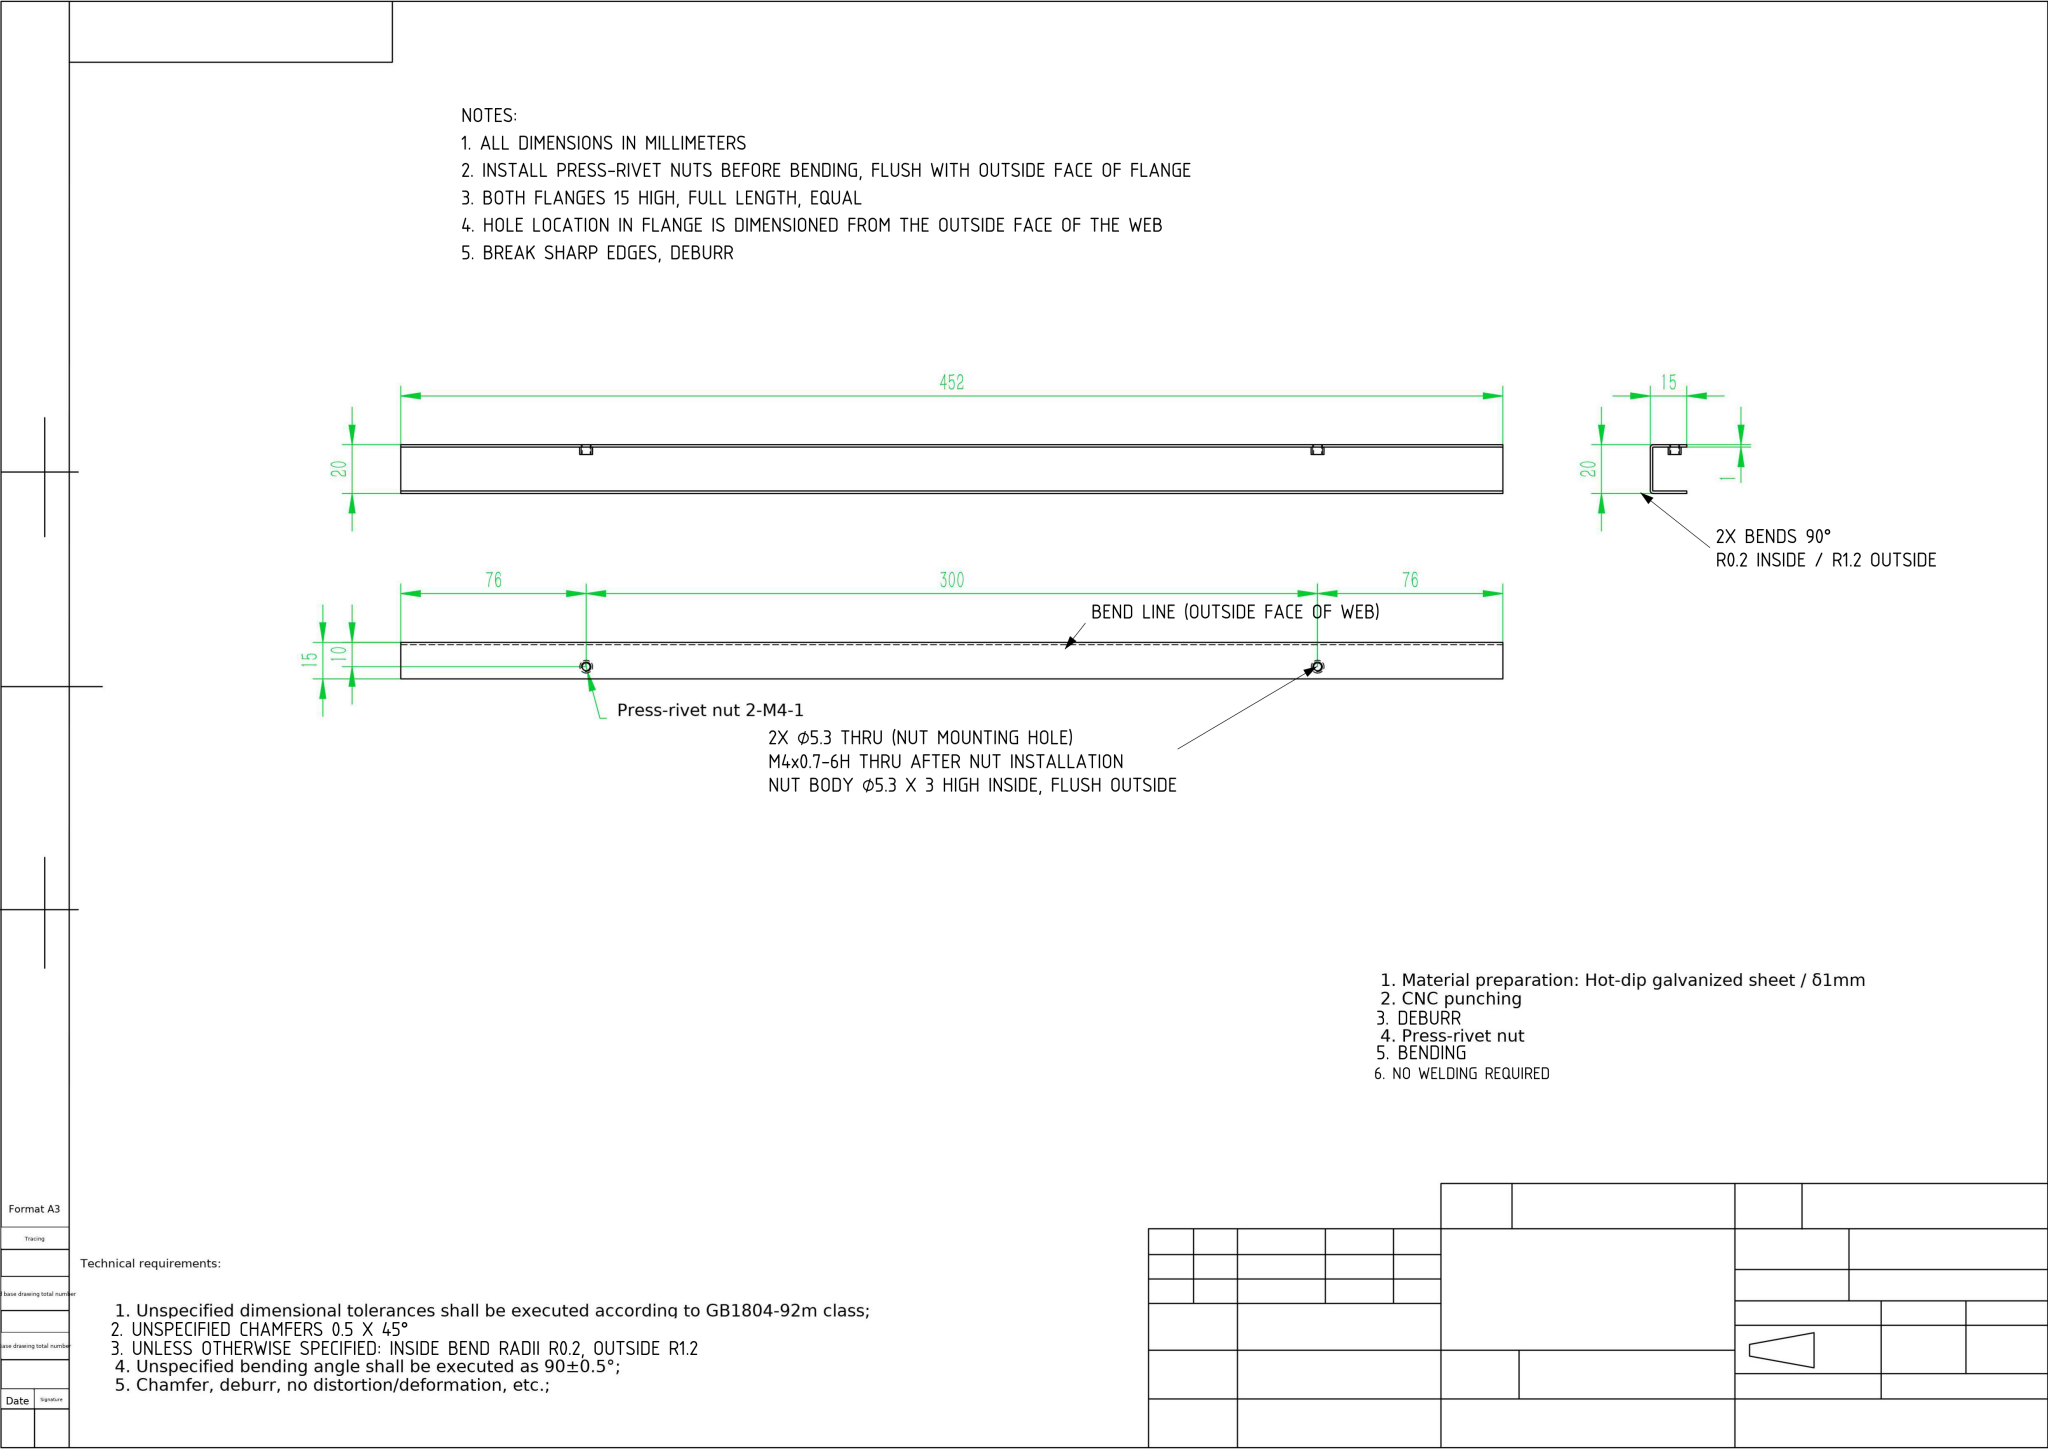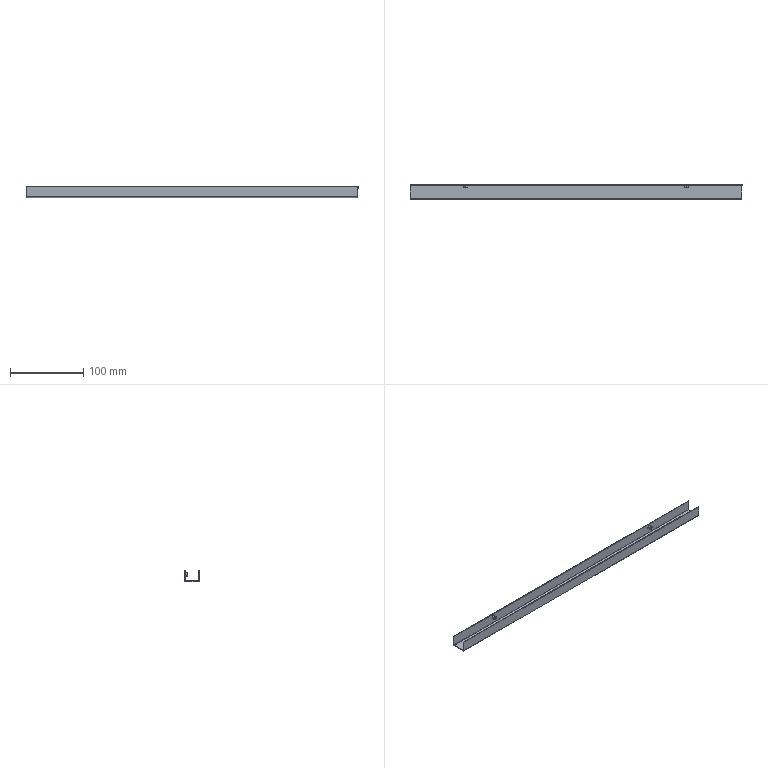Part | NX | mm | 1 solid | 32 faces | box 452 x 20 x 15 mm | volume 21488 mm3 | plane 20 | cylinder 12 | commonest cylinder face diameters 3.3 x4 5.3 x4 2.4 x2 0.4 x2
STEP:
#1=COLOUR_RGB('',0.7529,0.7529,0.7529);
#2=FILL_AREA_STYLE_COLOUR('',#1);
#3=FILL_AREA_STYLE('',(#2));
#4=SURFACE_STYLE_FILL_AREA(#3);
#5=SURFACE_SIDE_STYLE('',(#4));
#6=SURFACE_STYLE_USAGE(.BOTH.,#5);
#7=PRESENTATION_STYLE_ASSIGNMENT((#6));
#8=CARTESIAN_POINT('',(150.,6.,8.35));
#9=VERTEX_POINT('',#8);
#10=CARTESIAN_POINT('',(150.,10.,8.35));
#11=VERTEX_POINT('',#10);
#12=CARTESIAN_POINT('',(150.,10.,8.35));
#13=DIRECTION('',(-0.,1.,-0.));
#14=VECTOR('',#13,1000.);
#15=LINE('',#12,#14);
#16=EDGE_CURVE('',#9,#11,#15,.T.);
#17=ORIENTED_EDGE('',*,*,#16,.F.);
#18=CARTESIAN_POINT('',(150.,6.,11.65));
#19=VERTEX_POINT('',#18);
#20=CARTESIAN_POINT('',(150.,6.,10.));
#21=DIRECTION('',(-0.,1.,-0.));
#22=DIRECTION('',(0.,0.,1.));
#23=AXIS2_PLACEMENT_3D('',#20,#21,#22);
#24=CIRCLE('',#23,1.65);
#25=EDGE_CURVE('',#19,#9,#24,.T.);
#26=ORIENTED_EDGE('',*,*,#25,.F.);
#27=CARTESIAN_POINT('',(150.,10.,11.65));
#28=VERTEX_POINT('',#27);
#29=CARTESIAN_POINT('',(150.,10.,11.65));
#30=DIRECTION('',(-0.,1.,-0.));
#31=VECTOR('',#30,1000.);
#32=LINE('',#29,#31);
#33=EDGE_CURVE('',#19,#28,#32,.T.);
#34=ORIENTED_EDGE('',*,*,#33,.T.);
#35=CARTESIAN_POINT('',(150.,10.,10.));
#36=DIRECTION('',(-0.,1.,-0.));
#37=DIRECTION('',(0.,0.,1.));
#38=AXIS2_PLACEMENT_3D('',#35,#36,#37);
#39=CIRCLE('',#38,1.65);
#40=EDGE_CURVE('',#28,#11,#39,.T.);
#41=ORIENTED_EDGE('',*,*,#40,.T.);
#42=EDGE_LOOP('',(#17,#26,#34,#41));
#43=FACE_OUTER_BOUND('',#42,.T.);
#44=CARTESIAN_POINT('',(150.,10.,10.));
#45=DIRECTION('',(-0.,1.,-0.));
#46=DIRECTION('',(0.,0.,1.));
#47=AXIS2_PLACEMENT_3D('',#44,#45,#46);
#48=CYLINDRICAL_SURFACE('',#47,1.65);
#49=ADVANCED_FACE('',(#43),#48,.F.);
#50=STYLED_ITEM('',(#7),#49);
#51=PRESENTATION_LAYER_ASSIGNMENT('','',(#50));
#52=COLOUR_RGB('',0.7529,0.7529,0.7529);
#53=FILL_AREA_STYLE_COLOUR('',#52);
#54=FILL_AREA_STYLE('',(#53));
#55=SURFACE_STYLE_FILL_AREA(#54);
#56=SURFACE_SIDE_STYLE('',(#55));
#57=SURFACE_STYLE_USAGE(.BOTH.,#56);
#58=PRESENTATION_STYLE_ASSIGNMENT((#57));
#59=CARTESIAN_POINT('',(-150.,6.,8.35));
#60=VERTEX_POINT('',#59);
#61=CARTESIAN_POINT('',(-150.,10.,8.35));
#62=VERTEX_POINT('',#61);
#63=CARTESIAN_POINT('',(-150.,10.,8.35));
#64=DIRECTION('',(-0.,1.,-0.));
#65=VECTOR('',#64,1000.);
#66=LINE('',#63,#65);
#67=EDGE_CURVE('',#60,#62,#66,.T.);
#68=ORIENTED_EDGE('',*,*,#67,.F.);
#69=CARTESIAN_POINT('',(-150.,6.,11.65));
#70=VERTEX_POINT('',#69);
#71=CARTESIAN_POINT('',(-150.,6.,10.));
#72=DIRECTION('',(-0.,1.,-0.));
#73=DIRECTION('',(0.,0.,1.));
#74=AXIS2_PLACEMENT_3D('',#71,#72,#73);
#75=CIRCLE('',#74,1.65);
#76=EDGE_CURVE('',#70,#60,#75,.T.);
#77=ORIENTED_EDGE('',*,*,#76,.F.);
#78=CARTESIAN_POINT('',(-150.,10.,11.65));
#79=VERTEX_POINT('',#78);
#80=CARTESIAN_POINT('',(-150.,10.,11.65));
#81=DIRECTION('',(-0.,1.,-0.));
#82=VECTOR('',#81,1000.);
#83=LINE('',#80,#82);
#84=EDGE_CURVE('',#70,#79,#83,.T.);
#85=ORIENTED_EDGE('',*,*,#84,.T.);
#86=CARTESIAN_POINT('',(-150.,10.,10.));
#87=DIRECTION('',(-0.,1.,-0.));
#88=DIRECTION('',(0.,0.,1.));
#89=AXIS2_PLACEMENT_3D('',#86,#87,#88);
#90=CIRCLE('',#89,1.65);
#91=EDGE_CURVE('',#79,#62,#90,.T.);
#92=ORIENTED_EDGE('',*,*,#91,.T.);
#93=EDGE_LOOP('',(#68,#77,#85,#92));
#94=FACE_OUTER_BOUND('',#93,.T.);
#95=CARTESIAN_POINT('',(-150.,10.,10.));
#96=DIRECTION('',(-0.,1.,-0.));
#97=DIRECTION('',(0.,0.,1.));
#98=AXIS2_PLACEMENT_3D('',#95,#96,#97);
#99=CYLINDRICAL_SURFACE('',#98,1.65);
#100=ADVANCED_FACE('',(#94),#99,.F.);
#101=STYLED_ITEM('',(#58),#100);
#102=(LENGTH_UNIT()NAMED_UNIT(*)SI_UNIT(.MILLI.,.METRE.));
#103=UNCERTAINTY_MEASURE_WITH_UNIT(LENGTH_MEASURE(0.00001),#102,'','');
#104=(NAMED_UNIT(*)PLANE_ANGLE_UNIT()SI_UNIT($,.RADIAN.));
#105=(NAMED_UNIT(*)SI_UNIT($,.STERADIAN.)SOLID_ANGLE_UNIT());
#106=(GEOMETRIC_REPRESENTATION_CONTEXT(3)GLOBAL_UNCERTAINTY_ASSIGNED_CONTEXT((#103))GLOBAL_UNIT_ASSIGNED_CONTEXT((#102,#104,#105))REPRESENTATION_CONTEXT('',''));
#107=MECHANICAL_DESIGN_GEOMETRIC_PRESENTATION_REPRESENTATION('',(#101),#106);
#108=COLOUR_RGB('',0.7529,0.7529,0.7529);
#109=FILL_AREA_STYLE_COLOUR('',#108);
#110=FILL_AREA_STYLE('',(#109));
#111=SURFACE_STYLE_FILL_AREA(#110);
#112=SURFACE_SIDE_STYLE('',(#111));
#113=SURFACE_STYLE_USAGE(.BOTH.,#112);
#114=PRESENTATION_STYLE_ASSIGNMENT((#113));
#115=CARTESIAN_POINT('',(-150.,6.,10.));
#116=DIRECTION('',(-0.,1.,-0.));
#117=DIRECTION('',(0.,0.,1.));
#118=AXIS2_PLACEMENT_3D('',#115,#116,#117);
#119=CIRCLE('',#118,1.65);
#120=EDGE_CURVE('',#60,#70,#119,.T.);
#121=ORIENTED_EDGE('',*,*,#120,.F.);
#122=ORIENTED_EDGE('',*,*,#67,.T.);
#123=CARTESIAN_POINT('',(-150.,10.,10.));
#124=DIRECTION('',(-0.,1.,-0.));
#125=DIRECTION('',(0.,0.,1.));
#126=AXIS2_PLACEMENT_3D('',#123,#124,#125);
#127=CIRCLE('',#126,1.65);
#128=EDGE_CURVE('',#62,#79,#127,.T.);
#129=ORIENTED_EDGE('',*,*,#128,.T.);
#130=ORIENTED_EDGE('',*,*,#84,.F.);
#131=EDGE_LOOP('',(#121,#122,#129,#130));
#132=FACE_OUTER_BOUND('',#131,.T.);
#133=CARTESIAN_POINT('',(-150.,10.,10.));
#134=DIRECTION('',(-0.,1.,-0.));
#135=DIRECTION('',(0.,0.,1.));
#136=AXIS2_PLACEMENT_3D('',#133,#134,#135);
#137=CYLINDRICAL_SURFACE('',#136,1.65);
#138=ADVANCED_FACE('',(#132),#137,.F.);
#139=STYLED_ITEM('',(#114),#138);
#140=PRESENTATION_LAYER_ASSIGNMENT('','',(#139));
#141=COLOUR_RGB('',0.7529,0.7529,0.7529);
#142=FILL_AREA_STYLE_COLOUR('',#141);
#143=FILL_AREA_STYLE('',(#142));
#144=SURFACE_STYLE_FILL_AREA(#143);
#145=SURFACE_SIDE_STYLE('',(#144));
#146=SURFACE_STYLE_USAGE(.BOTH.,#145);
#147=PRESENTATION_STYLE_ASSIGNMENT((#146));
#148=CARTESIAN_POINT('',(150.,6.,10.));
#149=DIRECTION('',(-0.,1.,-0.));
#150=DIRECTION('',(0.,0.,1.));
#151=AXIS2_PLACEMENT_3D('',#148,#149,#150);
#152=CIRCLE('',#151,1.65);
#153=EDGE_CURVE('',#9,#19,#152,.T.);
#154=ORIENTED_EDGE('',*,*,#153,.F.);
#155=ORIENTED_EDGE('',*,*,#16,.T.);
#156=CARTESIAN_POINT('',(150.,10.,10.));
#157=DIRECTION('',(-0.,1.,-0.));
#158=DIRECTION('',(0.,0.,1.));
#159=AXIS2_PLACEMENT_3D('',#156,#157,#158);
#160=CIRCLE('',#159,1.65);
#161=EDGE_CURVE('',#11,#28,#160,.T.);
#162=ORIENTED_EDGE('',*,*,#161,.T.);
#163=ORIENTED_EDGE('',*,*,#33,.F.);
#164=EDGE_LOOP('',(#154,#155,#162,#163));
#165=FACE_OUTER_BOUND('',#164,.T.);
#166=CARTESIAN_POINT('',(150.,10.,10.));
#167=DIRECTION('',(-0.,1.,-0.));
#168=DIRECTION('',(0.,0.,1.));
#169=AXIS2_PLACEMENT_3D('',#166,#167,#168);
#170=CYLINDRICAL_SURFACE('',#169,1.65);
#171=ADVANCED_FACE('',(#165),#170,.F.);
#172=CARTESIAN_POINT('',(150.,6.,7.35));
#173=VERTEX_POINT('',#172);
#174=CARTESIAN_POINT('',(150.,6.,12.65));
#175=VERTEX_POINT('',#174);
#176=CARTESIAN_POINT('',(150.,6.,10.));
#177=DIRECTION('',(0.,-1.,0.));
#178=DIRECTION('',(0.,0.,1.));
#179=AXIS2_PLACEMENT_3D('',#176,#177,#178);
#180=CIRCLE('',#179,2.65);
#181=EDGE_CURVE('',#173,#175,#180,.T.);
#182=ORIENTED_EDGE('',*,*,#181,.F.);
#183=CARTESIAN_POINT('',(150.,9.,7.35));
#184=VERTEX_POINT('',#183);
#185=CARTESIAN_POINT('',(150.,6.,7.35));
#186=DIRECTION('',(-0.,1.,-0.));
#187=VECTOR('',#186,1000.);
#188=LINE('',#185,#187);
#189=EDGE_CURVE('',#173,#184,#188,.T.);
#190=ORIENTED_EDGE('',*,*,#189,.T.);
#191=CARTESIAN_POINT('',(150.,9.,12.65));
#192=VERTEX_POINT('',#191);
#193=CARTESIAN_POINT('',(150.,9.,10.));
#194=DIRECTION('',(0.,-1.,0.));
#195=DIRECTION('',(0.,0.,1.));
#196=AXIS2_PLACEMENT_3D('',#193,#194,#195);
#197=CIRCLE('',#196,2.65);
#198=EDGE_CURVE('',#184,#192,#197,.T.);
#199=ORIENTED_EDGE('',*,*,#198,.T.);
#200=CARTESIAN_POINT('',(150.,6.,12.65));
#201=DIRECTION('',(-0.,1.,-0.));
#202=VECTOR('',#201,1000.);
#203=LINE('',#200,#202);
#204=EDGE_CURVE('',#175,#192,#203,.T.);
#205=ORIENTED_EDGE('',*,*,#204,.F.);
#206=EDGE_LOOP('',(#182,#190,#199,#205));
#207=FACE_OUTER_BOUND('',#206,.T.);
#208=CARTESIAN_POINT('',(150.,6.,10.));
#209=DIRECTION('',(-0.,1.,-0.));
#210=DIRECTION('',(0.,0.,1.));
#211=AXIS2_PLACEMENT_3D('',#208,#209,#210);
#212=CYLINDRICAL_SURFACE('',#211,2.65);
#213=ADVANCED_FACE('',(#207),#212,.T.);
#214=CARTESIAN_POINT('',(-150.,6.,12.65));
#215=VERTEX_POINT('',#214);
#216=CARTESIAN_POINT('',(-150.,6.,7.35));
#217=VERTEX_POINT('',#216);
#218=CARTESIAN_POINT('',(-150.,6.,10.));
#219=DIRECTION('',(-0.,1.,-0.));
#220=DIRECTION('',(0.,0.,1.));
#221=AXIS2_PLACEMENT_3D('',#218,#219,#220);
#222=CIRCLE('',#221,2.65);
#223=EDGE_CURVE('',#215,#217,#222,.T.);
#224=ORIENTED_EDGE('',*,*,#223,.T.);
#225=CARTESIAN_POINT('',(-150.,9.,7.35));
#226=VERTEX_POINT('',#225);
#227=CARTESIAN_POINT('',(-150.,6.,7.35));
#228=DIRECTION('',(-0.,1.,-0.));
#229=VECTOR('',#228,1000.);
#230=LINE('',#227,#229);
#231=EDGE_CURVE('',#217,#226,#230,.T.);
#232=ORIENTED_EDGE('',*,*,#231,.T.);
#233=CARTESIAN_POINT('',(-150.,9.,12.65));
#234=VERTEX_POINT('',#233);
#235=CARTESIAN_POINT('',(-150.,9.,10.));
#236=DIRECTION('',(-0.,1.,-0.));
#237=DIRECTION('',(0.,0.,1.));
#238=AXIS2_PLACEMENT_3D('',#235,#236,#237);
#239=CIRCLE('',#238,2.65);
#240=EDGE_CURVE('',#234,#226,#239,.T.);
#241=ORIENTED_EDGE('',*,*,#240,.F.);
#242=CARTESIAN_POINT('',(-150.,6.,12.65));
#243=DIRECTION('',(-0.,1.,-0.));
#244=VECTOR('',#243,1000.);
#245=LINE('',#242,#244);
#246=EDGE_CURVE('',#215,#234,#245,.T.);
#247=ORIENTED_EDGE('',*,*,#246,.F.);
#248=EDGE_LOOP('',(#224,#232,#241,#247));
#249=FACE_OUTER_BOUND('',#248,.T.);
#250=CARTESIAN_POINT('',(-150.,6.,10.));
#251=DIRECTION('',(-0.,1.,-0.));
#252=DIRECTION('',(0.,0.,1.));
#253=AXIS2_PLACEMENT_3D('',#250,#251,#252);
#254=CYLINDRICAL_SURFACE('',#253,2.65);
#255=ADVANCED_FACE('',(#249),#254,.T.);
#256=CARTESIAN_POINT('',(226.,9.,1.2));
#257=VERTEX_POINT('',#256);
#258=CARTESIAN_POINT('',(-226.,9.,1.2));
#259=VERTEX_POINT('',#258);
#260=CARTESIAN_POINT('',(226.,9.,1.2));
#261=DIRECTION('',(-1.,0.,0.));
#262=VECTOR('',#261,1000.);
#263=LINE('',#260,#262);
#264=EDGE_CURVE('',#257,#259,#263,.T.);
#265=ORIENTED_EDGE('',*,*,#264,.F.);
#266=CARTESIAN_POINT('',(226.,9.,15.));
#267=VERTEX_POINT('',#266);
#268=CARTESIAN_POINT('',(226.,9.,-0.));
#269=DIRECTION('',(-0.,0.,1.));
#270=VECTOR('',#269,1000.);
#271=LINE('',#268,#270);
#272=EDGE_CURVE('',#257,#267,#271,.T.);
#273=ORIENTED_EDGE('',*,*,#272,.T.);
#274=CARTESIAN_POINT('',(-226.,9.,15.));
#275=VERTEX_POINT('',#274);
#276=CARTESIAN_POINT('',(0.,9.,15.));
#277=DIRECTION('',(-1.,0.,0.));
#278=VECTOR('',#277,1000.);
#279=LINE('',#276,#278);
#280=EDGE_CURVE('',#267,#275,#279,.T.);
#281=ORIENTED_EDGE('',*,*,#280,.T.);
#282=CARTESIAN_POINT('',(-226.,9.,0.));
#283=DIRECTION('',(0.,-0.,-1.));
#284=VECTOR('',#283,1000.);
#285=LINE('',#282,#284);
#286=EDGE_CURVE('',#275,#259,#285,.T.);
#287=ORIENTED_EDGE('',*,*,#286,.T.);
#288=EDGE_LOOP('',(#265,#273,#281,#287));
#289=FACE_OUTER_BOUND('',#288,.T.);
#290=ORIENTED_EDGE('',*,*,#240,.T.);
#291=CARTESIAN_POINT('',(-150.,9.,10.));
#292=DIRECTION('',(-0.,1.,-0.));
#293=DIRECTION('',(0.,0.,1.));
#294=AXIS2_PLACEMENT_3D('',#291,#292,#293);
#295=CIRCLE('',#294,2.65);
#296=EDGE_CURVE('',#226,#234,#295,.T.);
#297=ORIENTED_EDGE('',*,*,#296,.T.);
#298=EDGE_LOOP('',(#290,#297));
#299=FACE_BOUND('',#298,.T.);
#300=CARTESIAN_POINT('',(150.,9.,10.));
#301=DIRECTION('',(0.,-1.,0.));
#302=DIRECTION('',(0.,0.,1.));
#303=AXIS2_PLACEMENT_3D('',#300,#301,#302);
#304=CIRCLE('',#303,2.65);
#305=EDGE_CURVE('',#192,#184,#304,.T.);
#306=ORIENTED_EDGE('',*,*,#305,.F.);
#307=ORIENTED_EDGE('',*,*,#198,.F.);
#308=EDGE_LOOP('',(#306,#307));
#309=FACE_BOUND('',#308,.T.);
#310=CARTESIAN_POINT('',(-0.,9.,0.));
#311=DIRECTION('',(-0.,1.,-0.));
#312=DIRECTION('',(-0.,0.,1.));
#313=AXIS2_PLACEMENT_3D('',#310,#311,#312);
#314=PLANE('',#313);
#315=ADVANCED_FACE('',(#289,#299,#309),#314,.F.);
#316=CARTESIAN_POINT('',(-226.,-8.8,1.));
#317=VERTEX_POINT('',#316);
#318=CARTESIAN_POINT('',(-226.,-8.8,0.));
#319=VERTEX_POINT('',#318);
#320=CARTESIAN_POINT('',(-226.,-8.8,1.));
#321=DIRECTION('',(0.,0.,-1.));
#322=VECTOR('',#321,1000.);
#323=LINE('',#320,#322);
#324=EDGE_CURVE('',#317,#319,#323,.T.);
#325=ORIENTED_EDGE('',*,*,#324,.F.);
#326=CARTESIAN_POINT('',(-226.,8.8,1.));
#327=VERTEX_POINT('',#326);
#328=CARTESIAN_POINT('',(-226.,10.,1.));
#329=DIRECTION('',(0.,-1.,-0.));
#330=VECTOR('',#329,1000.);
#331=LINE('',#328,#330);
#332=EDGE_CURVE('',#327,#317,#331,.T.);
#333=ORIENTED_EDGE('',*,*,#332,.F.);
#334=CARTESIAN_POINT('',(-226.,8.8,0.));
#335=VERTEX_POINT('',#334);
#336=CARTESIAN_POINT('',(-226.,8.8,1.));
#337=DIRECTION('',(0.,-0.,-1.));
#338=VECTOR('',#337,1000.);
#339=LINE('',#336,#338);
#340=EDGE_CURVE('',#327,#335,#339,.T.);
#341=ORIENTED_EDGE('',*,*,#340,.T.);
#342=CARTESIAN_POINT('',(-226.,10.,0.));
#343=DIRECTION('',(0.,-1.,-0.));
#344=VECTOR('',#343,1000.);
#345=LINE('',#342,#344);
#346=EDGE_CURVE('',#335,#319,#345,.T.);
#347=ORIENTED_EDGE('',*,*,#346,.T.);
#348=EDGE_LOOP('',(#325,#333,#341,#347));
#349=FACE_OUTER_BOUND('',#348,.T.);
#350=CARTESIAN_POINT('',(-226.,10.,1.));
#351=DIRECTION('',(1.,-0.,0.));
#352=DIRECTION('',(0.,-0.,-1.));
#353=AXIS2_PLACEMENT_3D('',#350,#351,#352);
#354=PLANE('',#353);
#355=ADVANCED_FACE('',(#349),#354,.F.);
#356=CARTESIAN_POINT('',(226.,-8.8,1.));
#357=VERTEX_POINT('',#356);
#358=CARTESIAN_POINT('',(226.,-8.8,-0.));
#359=VERTEX_POINT('',#358);
#360=CARTESIAN_POINT('',(226.,-8.8,1.));
#361=DIRECTION('',(0.,0.,-1.));
#362=VECTOR('',#361,1000.);
#363=LINE('',#360,#362);
#364=EDGE_CURVE('',#357,#359,#363,.T.);
#365=ORIENTED_EDGE('',*,*,#364,.T.);
#366=CARTESIAN_POINT('',(226.,8.8,-0.));
#367=VERTEX_POINT('',#366);
#368=CARTESIAN_POINT('',(226.,10.,-0.));
#369=DIRECTION('',(-0.,1.,0.));
#370=VECTOR('',#369,1000.);
#371=LINE('',#368,#370);
#372=EDGE_CURVE('',#359,#367,#371,.T.);
#373=ORIENTED_EDGE('',*,*,#372,.T.);
#374=CARTESIAN_POINT('',(226.,8.8,1.));
#375=VERTEX_POINT('',#374);
#376=CARTESIAN_POINT('',(226.,8.8,1.));
#377=DIRECTION('',(0.,-0.,-1.));
#378=VECTOR('',#377,1000.);
#379=LINE('',#376,#378);
#380=EDGE_CURVE('',#375,#367,#379,.T.);
#381=ORIENTED_EDGE('',*,*,#380,.F.);
#382=CARTESIAN_POINT('',(226.,10.,1.));
#383=DIRECTION('',(-0.,1.,0.));
#384=VECTOR('',#383,1000.);
#385=LINE('',#382,#384);
#386=EDGE_CURVE('',#357,#375,#385,.T.);
#387=ORIENTED_EDGE('',*,*,#386,.F.);
#388=EDGE_LOOP('',(#365,#373,#381,#387));
#389=FACE_OUTER_BOUND('',#388,.T.);
#390=CARTESIAN_POINT('',(226.,10.,1.));
#391=DIRECTION('',(-1.,0.,-0.));
#392=DIRECTION('',(-0.,0.,1.));
#393=AXIS2_PLACEMENT_3D('',#390,#391,#392);
#394=PLANE('',#393);
#395=ADVANCED_FACE('',(#389),#394,.F.);
#396=CARTESIAN_POINT('',(226.,-8.8,1.));
#397=DIRECTION('',(-1.,0.,0.));
#398=VECTOR('',#397,1000.);
#399=LINE('',#396,#398);
#400=EDGE_CURVE('',#357,#317,#399,.T.);
#401=ORIENTED_EDGE('',*,*,#400,.F.);
#402=ORIENTED_EDGE('',*,*,#386,.T.);
#403=CARTESIAN_POINT('',(-226.,8.8,1.));
#404=DIRECTION('',(1.,-0.,-0.));
#405=VECTOR('',#404,1000.);
#406=LINE('',#403,#405);
#407=EDGE_CURVE('',#327,#375,#406,.T.);
#408=ORIENTED_EDGE('',*,*,#407,.F.);
#409=ORIENTED_EDGE('',*,*,#332,.T.);
#410=EDGE_LOOP('',(#401,#402,#408,#409));
#411=FACE_OUTER_BOUND('',#410,.T.);
#412=CARTESIAN_POINT('',(0.,0.,1.));
#413=DIRECTION('',(-0.,-0.,-1.));
#414=DIRECTION('',(-1.,0.,0.));
#415=AXIS2_PLACEMENT_3D('',#412,#413,#414);
#416=PLANE('',#415);
#417=ADVANCED_FACE('',(#411),#416,.F.);
#418=ORIENTED_EDGE('',*,*,#372,.F.);
#419=CARTESIAN_POINT('',(226.,-8.8,-0.));
#420=DIRECTION('',(-1.,0.,0.));
#421=VECTOR('',#420,1000.);
#422=LINE('',#419,#421);
#423=EDGE_CURVE('',#359,#319,#422,.T.);
#424=ORIENTED_EDGE('',*,*,#423,.T.);
#425=ORIENTED_EDGE('',*,*,#346,.F.);
#426=CARTESIAN_POINT('',(-226.,8.8,0.));
#427=DIRECTION('',(1.,-0.,-0.));
#428=VECTOR('',#427,1000.);
#429=LINE('',#426,#428);
#430=EDGE_CURVE('',#335,#367,#429,.T.);
#431=ORIENTED_EDGE('',*,*,#430,.T.);
#432=EDGE_LOOP('',(#418,#424,#425,#431));
#433=FACE_OUTER_BOUND('',#432,.T.);
#434=CARTESIAN_POINT('',(0.,0.,0.));
#435=DIRECTION('',(-0.,-0.,-1.));
#436=DIRECTION('',(-1.,0.,0.));
#437=AXIS2_PLACEMENT_3D('',#434,#435,#436);
#438=PLANE('',#437);
#439=ADVANCED_FACE('',(#433),#438,.T.);
#440=CARTESIAN_POINT('',(226.,10.,1.2));
#441=VERTEX_POINT('',#440);
#442=CARTESIAN_POINT('',(226.,10.,1.2));
#443=DIRECTION('',(-0.,1.,-0.));
#444=VECTOR('',#443,1000.);
#445=LINE('',#442,#444);
#446=EDGE_CURVE('',#257,#441,#445,.T.);
#447=ORIENTED_EDGE('',*,*,#446,.F.);
#448=CARTESIAN_POINT('',(226.,8.8,1.2));
#449=DIRECTION('',(1.,-0.,-0.));
#450=DIRECTION('',(0.,0.,1.));
#451=AXIS2_PLACEMENT_3D('',#448,#449,#450);
#452=CIRCLE('',#451,0.2);
#453=EDGE_CURVE('',#375,#257,#452,.T.);
#454=ORIENTED_EDGE('',*,*,#453,.F.);
#455=ORIENTED_EDGE('',*,*,#380,.T.);
#456=CARTESIAN_POINT('',(226.,8.8,1.2));
#457=DIRECTION('',(1.,-0.,-0.));
#458=DIRECTION('',(0.,0.,1.));
#459=AXIS2_PLACEMENT_3D('',#456,#457,#458);
#460=CIRCLE('',#459,1.2);
#461=EDGE_CURVE('',#367,#441,#460,.T.);
#462=ORIENTED_EDGE('',*,*,#461,.T.);
#463=EDGE_LOOP('',(#447,#454,#455,#462));
#464=FACE_OUTER_BOUND('',#463,.T.);
#465=CARTESIAN_POINT('',(226.,8.8,1.2));
#466=DIRECTION('',(1.,-0.,0.));
#467=DIRECTION('',(0.,-0.,-1.));
#468=AXIS2_PLACEMENT_3D('',#465,#466,#467);
#469=PLANE('',#468);
#470=ADVANCED_FACE('',(#464),#469,.T.);
#471=CARTESIAN_POINT('',(-226.,8.8,1.2));
#472=DIRECTION('',(-1.,0.,0.));
#473=DIRECTION('',(0.,0.,1.));
#474=AXIS2_PLACEMENT_3D('',#471,#472,#473);
#475=CIRCLE('',#474,0.2);
#476=EDGE_CURVE('',#259,#327,#475,.T.);
#477=ORIENTED_EDGE('',*,*,#476,.F.);
#478=CARTESIAN_POINT('',(-226.,10.,1.2));
#479=VERTEX_POINT('',#478);
#480=CARTESIAN_POINT('',(-226.,9.,1.2));
#481=DIRECTION('',(-0.,1.,-0.));
#482=VECTOR('',#481,1000.);
#483=LINE('',#480,#482);
#484=EDGE_CURVE('',#259,#479,#483,.T.);
#485=ORIENTED_EDGE('',*,*,#484,.T.);
#486=CARTESIAN_POINT('',(-226.,8.8,1.2));
#487=DIRECTION('',(-1.,0.,0.));
#488=DIRECTION('',(0.,0.,1.));
#489=AXIS2_PLACEMENT_3D('',#486,#487,#488);
#490=CIRCLE('',#489,1.2);
#491=EDGE_CURVE('',#479,#335,#490,.T.);
#492=ORIENTED_EDGE('',*,*,#491,.T.);
#493=ORIENTED_EDGE('',*,*,#340,.F.);
#494=EDGE_LOOP('',(#477,#485,#492,#493));
#495=FACE_OUTER_BOUND('',#494,.T.);
#496=CARTESIAN_POINT('',(-226.,8.8,1.2));
#497=DIRECTION('',(1.,-0.,0.));
#498=DIRECTION('',(0.,-0.,-1.));
#499=AXIS2_PLACEMENT_3D('',#496,#497,#498);
#500=PLANE('',#499);
#501=ADVANCED_FACE('',(#495),#500,.F.);
#502=ORIENTED_EDGE('',*,*,#430,.F.);
#503=ORIENTED_EDGE('',*,*,#491,.F.);
#504=CARTESIAN_POINT('',(-0.,10.,1.2));
#505=DIRECTION('',(-1.,0.,0.));
#506=VECTOR('',#505,1000.);
#507=LINE('',#504,#506);
#508=EDGE_CURVE('',#441,#479,#507,.T.);
#509=ORIENTED_EDGE('',*,*,#508,.F.);
#510=ORIENTED_EDGE('',*,*,#461,.F.);
#511=EDGE_LOOP('',(#502,#503,#509,#510));
#512=FACE_OUTER_BOUND('',#511,.T.);
#513=CARTESIAN_POINT('',(-226.,8.8,1.2));
#514=DIRECTION('',(-1.,0.,0.));
#515=DIRECTION('',(0.,1.,-0.));
#516=AXIS2_PLACEMENT_3D('',#513,#514,#515);
#517=CYLINDRICAL_SURFACE('',#516,1.2);
#518=ADVANCED_FACE('',(#512),#517,.T.);
#519=ORIENTED_EDGE('',*,*,#407,.T.);
#520=ORIENTED_EDGE('',*,*,#453,.T.);
#521=ORIENTED_EDGE('',*,*,#264,.T.);
#522=ORIENTED_EDGE('',*,*,#476,.T.);
#523=EDGE_LOOP('',(#519,#520,#521,#522));
#524=FACE_OUTER_BOUND('',#523,.T.);
#525=CARTESIAN_POINT('',(-226.,8.8,1.2));
#526=DIRECTION('',(-1.,0.,0.));
#527=DIRECTION('',(0.,1.,-0.));
#528=AXIS2_PLACEMENT_3D('',#525,#526,#527);
#529=CYLINDRICAL_SURFACE('',#528,0.2);
#530=ADVANCED_FACE('',(#524),#529,.F.);
#531=CARTESIAN_POINT('',(-226.,10.,15.));
#532=VERTEX_POINT('',#531);
#533=CARTESIAN_POINT('',(-226.,10.,1.));
#534=DIRECTION('',(0.,-0.,-1.));
#535=VECTOR('',#534,1000.);
#536=LINE('',#533,#535);
#537=EDGE_CURVE('',#532,#479,#536,.T.);
#538=ORIENTED_EDGE('',*,*,#537,.T.);
#539=ORIENTED_EDGE('',*,*,#484,.F.);
#540=ORIENTED_EDGE('',*,*,#286,.F.);
#541=CARTESIAN_POINT('',(-226.,10.,15.));
#542=DIRECTION('',(0.,-1.,0.));
#543=VECTOR('',#542,1000.);
#544=LINE('',#541,#543);
#545=EDGE_CURVE('',#532,#275,#544,.T.);
#546=ORIENTED_EDGE('',*,*,#545,.F.);
#547=EDGE_LOOP('',(#538,#539,#540,#546));
#548=FACE_OUTER_BOUND('',#547,.T.);
#549=CARTESIAN_POINT('',(-226.,10.,1.));
#550=DIRECTION('',(-1.,-0.,0.));
#551=DIRECTION('',(0.,-1.,-0.));
#552=AXIS2_PLACEMENT_3D('',#549,#550,#551);
#553=PLANE('',#552);
#554=ADVANCED_FACE('',(#548),#553,.T.);
#555=ORIENTED_EDGE('',*,*,#272,.F.);
#556=ORIENTED_EDGE('',*,*,#446,.T.);
#557=CARTESIAN_POINT('',(226.,10.,15.));
#558=VERTEX_POINT('',#557);
#559=CARTESIAN_POINT('',(226.,10.,15.));
#560=DIRECTION('',(-0.,0.,1.));
#561=VECTOR('',#560,1000.);
#562=LINE('',#559,#561);
#563=EDGE_CURVE('',#441,#558,#562,.T.);
#564=ORIENTED_EDGE('',*,*,#563,.T.);
#565=CARTESIAN_POINT('',(226.,10.,15.));
#566=DIRECTION('',(0.,-1.,0.));
#567=VECTOR('',#566,1000.);
#568=LINE('',#565,#567);
#569=EDGE_CURVE('',#558,#267,#568,.T.);
#570=ORIENTED_EDGE('',*,*,#569,.T.);
#571=EDGE_LOOP('',(#555,#556,#564,#570));
#572=FACE_OUTER_BOUND('',#571,.T.);
#573=CARTESIAN_POINT('',(226.,10.,15.));
#574=DIRECTION('',(1.,0.,-0.));
#575=DIRECTION('',(-0.,1.,0.));
#576=AXIS2_PLACEMENT_3D('',#573,#574,#575);
#577=PLANE('',#576);
#578=ADVANCED_FACE('',(#572),#577,.T.);
#579=ORIENTED_EDGE('',*,*,#40,.F.);
#580=ORIENTED_EDGE('',*,*,#161,.F.);
#581=EDGE_LOOP('',(#579,#580));
#582=FACE_BOUND('',#581,.T.);
#583=ORIENTED_EDGE('',*,*,#563,.F.);
#584=ORIENTED_EDGE('',*,*,#508,.T.);
#585=ORIENTED_EDGE('',*,*,#537,.F.);
#586=CARTESIAN_POINT('',(-226.,10.,15.));
#587=DIRECTION('',(-1.,0.,0.));
#588=VECTOR('',#587,1000.);
#589=LINE('',#586,#588);
#590=EDGE_CURVE('',#558,#532,#589,.T.);
#591=ORIENTED_EDGE('',*,*,#590,.F.);
#592=EDGE_LOOP('',(#583,#584,#585,#591));
#593=FACE_OUTER_BOUND('',#592,.T.);
#594=ORIENTED_EDGE('',*,*,#91,.F.);
#595=ORIENTED_EDGE('',*,*,#128,.F.);
#596=EDGE_LOOP('',(#594,#595));
#597=FACE_BOUND('',#596,.T.);
#598=CARTESIAN_POINT('',(-0.,10.,-0.));
#599=DIRECTION('',(-0.,1.,-0.));
#600=DIRECTION('',(-0.,0.,1.));
#601=AXIS2_PLACEMENT_3D('',#598,#599,#600);
#602=PLANE('',#601);
#603=ADVANCED_FACE('',(#582,#593,#597),#602,.T.);
#604=ORIENTED_EDGE('',*,*,#280,.F.);
#605=ORIENTED_EDGE('',*,*,#569,.F.);
#606=ORIENTED_EDGE('',*,*,#590,.T.);
#607=ORIENTED_EDGE('',*,*,#545,.T.);
#608=EDGE_LOOP('',(#604,#605,#606,#607));
#609=FACE_OUTER_BOUND('',#608,.T.);
#610=CARTESIAN_POINT('',(-226.,10.,15.));
#611=DIRECTION('',(-0.,0.,1.));
#612=DIRECTION('',(0.,-1.,0.));
#613=AXIS2_PLACEMENT_3D('',#610,#611,#612);
#614=PLANE('',#613);
#615=ADVANCED_FACE('',(#609),#614,.T.);
#616=CARTESIAN_POINT('',(-226.,-9.,1.2));
#617=VERTEX_POINT('',#616);
#618=CARTESIAN_POINT('',(-226.,-10.,1.2));
#619=VERTEX_POINT('',#618);
#620=CARTESIAN_POINT('',(-226.,-10.,1.2));
#621=DIRECTION('',(0.,-1.,-0.));
#622=VECTOR('',#621,1000.);
#623=LINE('',#620,#622);
#624=EDGE_CURVE('',#617,#619,#623,.T.);
#625=ORIENTED_EDGE('',*,*,#624,.F.);
#626=CARTESIAN_POINT('',(-226.,-8.8,1.2));
#627=DIRECTION('',(-1.,0.,0.));
#628=DIRECTION('',(0.,0.,-1.));
#629=AXIS2_PLACEMENT_3D('',#626,#627,#628);
#630=CIRCLE('',#629,0.2);
#631=EDGE_CURVE('',#317,#617,#630,.T.);
#632=ORIENTED_EDGE('',*,*,#631,.F.);
#633=ORIENTED_EDGE('',*,*,#324,.T.);
#634=CARTESIAN_POINT('',(-226.,-8.8,1.2));
#635=DIRECTION('',(-1.,0.,0.));
#636=DIRECTION('',(0.,0.,-1.));
#637=AXIS2_PLACEMENT_3D('',#634,#635,#636);
#638=CIRCLE('',#637,1.2);
#639=EDGE_CURVE('',#319,#619,#638,.T.);
#640=ORIENTED_EDGE('',*,*,#639,.T.);
#641=EDGE_LOOP('',(#625,#632,#633,#640));
#642=FACE_OUTER_BOUND('',#641,.T.);
#643=CARTESIAN_POINT('',(-226.,-8.8,1.2));
#644=DIRECTION('',(-1.,0.,-0.));
#645=DIRECTION('',(-0.,0.,1.));
#646=AXIS2_PLACEMENT_3D('',#643,#644,#645);
#647=PLANE('',#646);
#648=ADVANCED_FACE('',(#642),#647,.T.);
#649=CARTESIAN_POINT('',(226.,-9.,1.2));
#650=VERTEX_POINT('',#649);
#651=CARTESIAN_POINT('',(226.,-8.8,1.2));
#652=DIRECTION('',(1.,-0.,-0.));
#653=DIRECTION('',(0.,0.,-1.));
#654=AXIS2_PLACEMENT_3D('',#651,#652,#653);
#655=CIRCLE('',#654,0.2);
#656=EDGE_CURVE('',#650,#357,#655,.T.);
#657=ORIENTED_EDGE('',*,*,#656,.F.);
#658=CARTESIAN_POINT('',(226.,-10.,1.2));
#659=VERTEX_POINT('',#658);
#660=CARTESIAN_POINT('',(226.,-9.,1.2));
#661=DIRECTION('',(0.,-1.,-0.));
#662=VECTOR('',#661,1000.);
#663=LINE('',#660,#662);
#664=EDGE_CURVE('',#650,#659,#663,.T.);
#665=ORIENTED_EDGE('',*,*,#664,.T.);
#666=CARTESIAN_POINT('',(226.,-8.8,1.2));
#667=DIRECTION('',(1.,-0.,-0.));
#668=DIRECTION('',(0.,0.,-1.));
#669=AXIS2_PLACEMENT_3D('',#666,#667,#668);
#670=CIRCLE('',#669,1.2);
#671=EDGE_CURVE('',#659,#359,#670,.T.);
#672=ORIENTED_EDGE('',*,*,#671,.T.);
#673=ORIENTED_EDGE('',*,*,#364,.F.);
#674=EDGE_LOOP('',(#657,#665,#672,#673));
#675=FACE_OUTER_BOUND('',#674,.T.);
#676=CARTESIAN_POINT('',(226.,-8.8,1.2));
#677=DIRECTION('',(-1.,0.,-0.));
#678=DIRECTION('',(-0.,0.,1.));
#679=AXIS2_PLACEMENT_3D('',#676,#677,#678);
#680=PLANE('',#679);
#681=ADVANCED_FACE('',(#675),#680,.F.);
#682=ORIENTED_EDGE('',*,*,#423,.F.);
#683=ORIENTED_EDGE('',*,*,#671,.F.);
#684=CARTESIAN_POINT('',(-226.,-10.,1.2));
#685=DIRECTION('',(-1.,0.,0.));
#686=VECTOR('',#685,1000.);
#687=LINE('',#684,#686);
#688=EDGE_CURVE('',#659,#619,#687,.T.);
#689=ORIENTED_EDGE('',*,*,#688,.T.);
#690=ORIENTED_EDGE('',*,*,#639,.F.);
#691=EDGE_LOOP('',(#682,#683,#689,#690));
#692=FACE_OUTER_BOUND('',#691,.T.);
#693=CARTESIAN_POINT('',(226.,-8.8,1.2));
#694=DIRECTION('',(1.,-0.,-0.));
#695=DIRECTION('',(0.,-1.,-0.));
#696=AXIS2_PLACEMENT_3D('',#693,#694,#695);
#697=CYLINDRICAL_SURFACE('',#696,1.2);
#698=ADVANCED_FACE('',(#692),#697,.T.);
#699=ORIENTED_EDGE('',*,*,#400,.T.);
#700=ORIENTED_EDGE('',*,*,#631,.T.);
#701=CARTESIAN_POINT('',(-226.,-9.,1.2));
#702=DIRECTION('',(1.,-0.,-0.));
#703=VECTOR('',#702,1000.);
#704=LINE('',#701,#703);
#705=EDGE_CURVE('',#617,#650,#704,.T.);
#706=ORIENTED_EDGE('',*,*,#705,.T.);
#707=ORIENTED_EDGE('',*,*,#656,.T.);
#708=EDGE_LOOP('',(#699,#700,#706,#707));
#709=FACE_OUTER_BOUND('',#708,.T.);
#710=CARTESIAN_POINT('',(226.,-8.8,1.2));
#711=DIRECTION('',(1.,-0.,-0.));
#712=DIRECTION('',(0.,-1.,-0.));
#713=AXIS2_PLACEMENT_3D('',#710,#711,#712);
#714=CYLINDRICAL_SURFACE('',#713,0.2);
#715=ADVANCED_FACE('',(#709),#714,.F.);
#716=CARTESIAN_POINT('',(-226.,-9.,15.));
#717=VERTEX_POINT('',#716);
#718=CARTESIAN_POINT('',(-226.,-9.,0.));
#719=DIRECTION('',(-0.,-0.,1.));
#720=VECTOR('',#719,1000.);
#721=LINE('',#718,#720);
#722=EDGE_CURVE('',#617,#717,#721,.T.);
#723=ORIENTED_EDGE('',*,*,#722,.F.);
#724=ORIENTED_EDGE('',*,*,#624,.T.);
#725=CARTESIAN_POINT('',(-226.,-10.,15.));
#726=VERTEX_POINT('',#725);
#727=CARTESIAN_POINT('',(-226.,-10.,1.));
#728=DIRECTION('',(-0.,-0.,1.));
#729=VECTOR('',#728,1000.);
#730=LINE('',#727,#729);
#731=EDGE_CURVE('',#619,#726,#730,.T.);
#732=ORIENTED_EDGE('',*,*,#731,.T.);
#733=CARTESIAN_POINT('',(-226.,-10.,15.));
#734=DIRECTION('',(-0.,1.,0.));
#735=VECTOR('',#734,1000.);
#736=LINE('',#733,#735);
#737=EDGE_CURVE('',#726,#717,#736,.T.);
#738=ORIENTED_EDGE('',*,*,#737,.T.);
#739=EDGE_LOOP('',(#723,#724,#732,#738));
#740=FACE_OUTER_BOUND('',#739,.T.);
#741=CARTESIAN_POINT('',(-226.,-10.,1.));
#742=DIRECTION('',(-1.,-0.,0.));
#743=DIRECTION('',(0.,-1.,-0.));
#744=AXIS2_PLACEMENT_3D('',#741,#742,#743);
#745=PLANE('',#744);
#746=ADVANCED_FACE('',(#740),#745,.T.);
#747=CARTESIAN_POINT('',(226.,-10.,15.));
#748=VERTEX_POINT('',#747);
#749=CARTESIAN_POINT('',(226.,-10.,15.));
#750=DIRECTION('',(0.,0.,-1.));
#751=VECTOR('',#750,1000.);
#752=LINE('',#749,#751);
#753=EDGE_CURVE('',#748,#659,#752,.T.);
#754=ORIENTED_EDGE('',*,*,#753,.T.);
#755=ORIENTED_EDGE('',*,*,#664,.F.);
#756=CARTESIAN_POINT('',(226.,-9.,15.));
#757=VERTEX_POINT('',#756);
#758=CARTESIAN_POINT('',(226.,-9.,-0.));
#759=DIRECTION('',(0.,0.,-1.));
#760=VECTOR('',#759,1000.);
#761=LINE('',#758,#760);
#762=EDGE_CURVE('',#757,#650,#761,.T.);
#763=ORIENTED_EDGE('',*,*,#762,.F.);
#764=CARTESIAN_POINT('',(226.,-10.,15.));
#765=DIRECTION('',(-0.,1.,0.));
#766=VECTOR('',#765,1000.);
#767=LINE('',#764,#766);
#768=EDGE_CURVE('',#748,#757,#767,.T.);
#769=ORIENTED_EDGE('',*,*,#768,.F.);
#770=EDGE_LOOP('',(#754,#755,#763,#769));
#771=FACE_OUTER_BOUND('',#770,.T.);
#772=CARTESIAN_POINT('',(226.,-10.,15.));
#773=DIRECTION('',(1.,0.,-0.));
#774=DIRECTION('',(-0.,1.,0.));
#775=AXIS2_PLACEMENT_3D('',#772,#773,#774);
#776=PLANE('',#775);
#777=ADVANCED_FACE('',(#771),#776,.T.);
#778=ORIENTED_EDGE('',*,*,#688,.F.);
#779=ORIENTED_EDGE('',*,*,#753,.F.);
#780=CARTESIAN_POINT('',(-226.,-10.,15.));
#781=DIRECTION('',(1.,-0.,-0.));
#782=VECTOR('',#781,1000.);
#783=LINE('',#780,#782);
#784=EDGE_CURVE('',#726,#748,#783,.T.);
#785=ORIENTED_EDGE('',*,*,#784,.F.);
#786=ORIENTED_EDGE('',*,*,#731,.F.);
#787=EDGE_LOOP('',(#778,#779,#785,#786));
#788=FACE_OUTER_BOUND('',#787,.T.);
#789=CARTESIAN_POINT('',(-0.,-10.,0.));
#790=DIRECTION('',(-0.,1.,0.));
#791=DIRECTION('',(-0.,-0.,1.));
#792=AXIS2_PLACEMENT_3D('',#789,#790,#791);
#793=PLANE('',#792);
#794=ADVANCED_FACE('',(#788),#793,.F.);
#795=ORIENTED_EDGE('',*,*,#762,.T.);
#796=ORIENTED_EDGE('',*,*,#705,.F.);
#797=ORIENTED_EDGE('',*,*,#722,.T.);
#798=CARTESIAN_POINT('',(0.,-9.,15.));
#799=DIRECTION('',(1.,-0.,-0.));
#800=VECTOR('',#799,1000.);
#801=LINE('',#798,#800);
#802=EDGE_CURVE('',#717,#757,#801,.T.);
#803=ORIENTED_EDGE('',*,*,#802,.T.);
#804=EDGE_LOOP('',(#795,#796,#797,#803));
#805=FACE_OUTER_BOUND('',#804,.T.);
#806=CARTESIAN_POINT('',(-0.,-9.,-0.));
#807=DIRECTION('',(-0.,1.,0.));
#808=DIRECTION('',(-0.,-0.,1.));
#809=AXIS2_PLACEMENT_3D('',#806,#807,#808);
#810=PLANE('',#809);
#811=ADVANCED_FACE('',(#805),#810,.T.);
#812=ORIENTED_EDGE('',*,*,#802,.F.);
#813=ORIENTED_EDGE('',*,*,#737,.F.);
#814=ORIENTED_EDGE('',*,*,#784,.T.);
#815=ORIENTED_EDGE('',*,*,#768,.T.);
#816=EDGE_LOOP('',(#812,#813,#814,#815));
#817=FACE_OUTER_BOUND('',#816,.T.);
#818=CARTESIAN_POINT('',(-226.,-10.,15.));
#819=DIRECTION('',(-0.,-0.,1.));
#820=DIRECTION('',(0.,-1.,-0.));
#821=AXIS2_PLACEMENT_3D('',#818,#819,#820);
#822=PLANE('',#821);
#823=ADVANCED_FACE('',(#817),#822,.T.);
#824=ORIENTED_EDGE('',*,*,#231,.F.);
#825=CARTESIAN_POINT('',(-150.,6.,10.));
#826=DIRECTION('',(-0.,1.,-0.));
#827=DIRECTION('',(0.,0.,1.));
#828=AXIS2_PLACEMENT_3D('',#825,#826,#827);
#829=CIRCLE('',#828,2.65);
#830=EDGE_CURVE('',#217,#215,#829,.T.);
#831=ORIENTED_EDGE('',*,*,#830,.T.);
#832=ORIENTED_EDGE('',*,*,#246,.T.);
#833=ORIENTED_EDGE('',*,*,#296,.F.);
#834=EDGE_LOOP('',(#824,#831,#832,#833));
#835=FACE_OUTER_BOUND('',#834,.T.);
#836=CARTESIAN_POINT('',(-150.,6.,10.));
#837=DIRECTION('',(-0.,1.,-0.));
#838=DIRECTION('',(0.,0.,1.));
#839=AXIS2_PLACEMENT_3D('',#836,#837,#838);
#840=CYLINDRICAL_SURFACE('',#839,2.65);
#841=ADVANCED_FACE('',(#835),#840,.T.);
#842=ORIENTED_EDGE('',*,*,#76,.T.);
#843=ORIENTED_EDGE('',*,*,#120,.T.);
#844=EDGE_LOOP('',(#842,#843));
#845=FACE_BOUND('',#844,.T.);
#846=ORIENTED_EDGE('',*,*,#223,.F.);
#847=ORIENTED_EDGE('',*,*,#830,.F.);
#848=EDGE_LOOP('',(#846,#847));
#849=FACE_OUTER_BOUND('',#848,.T.);
#850=CARTESIAN_POINT('',(-150.,6.,10.));
#851=DIRECTION('',(-0.,1.,-0.));
#852=DIRECTION('',(-0.,0.,1.));
#853=AXIS2_PLACEMENT_3D('',#850,#851,#852);
#854=PLANE('',#853);
#855=ADVANCED_FACE('',(#845,#849),#854,.F.);
#856=ORIENTED_EDGE('',*,*,#189,.F.);
#857=CARTESIAN_POINT('',(150.,6.,10.));
#858=DIRECTION('',(0.,-1.,0.));
#859=DIRECTION('',(0.,0.,1.));
#860=AXIS2_PLACEMENT_3D('',#857,#858,#859);
#861=CIRCLE('',#860,2.65);
#862=EDGE_CURVE('',#175,#173,#861,.T.);
#863=ORIENTED_EDGE('',*,*,#862,.F.);
#864=ORIENTED_EDGE('',*,*,#204,.T.);
#865=ORIENTED_EDGE('',*,*,#305,.T.);
#866=EDGE_LOOP('',(#856,#863,#864,#865));
#867=FACE_OUTER_BOUND('',#866,.T.);
#868=CARTESIAN_POINT('',(150.,6.,10.));
#869=DIRECTION('',(-0.,1.,-0.));
#870=DIRECTION('',(0.,0.,1.));
#871=AXIS2_PLACEMENT_3D('',#868,#869,#870);
#872=CYLINDRICAL_SURFACE('',#871,2.65);
#873=ADVANCED_FACE('',(#867),#872,.T.);
#874=ORIENTED_EDGE('',*,*,#25,.T.);
#875=ORIENTED_EDGE('',*,*,#153,.T.);
#876=EDGE_LOOP('',(#874,#875));
#877=FACE_BOUND('',#876,.T.);
#878=ORIENTED_EDGE('',*,*,#862,.T.);
#879=ORIENTED_EDGE('',*,*,#181,.T.);
#880=EDGE_LOOP('',(#878,#879));
#881=FACE_OUTER_BOUND('',#880,.T.);
#882=CARTESIAN_POINT('',(150.,6.,10.));
#883=DIRECTION('',(-0.,1.,-0.));
#884=DIRECTION('',(-0.,0.,1.));
#885=AXIS2_PLACEMENT_3D('',#882,#883,#884);
#886=PLANE('',#885);
#887=ADVANCED_FACE('',(#877,#881),#886,.F.);
#888=CLOSED_SHELL('',(#171,#213,#138,#255,#315,#355,#395,#417,#439,#470,#501,#518,#530,#554,#578,#603,#615,#648,#681,#698,#715,#746,#777,#794,#811,#823,#841,#855,#100,#873,#887,#49));
#889=MANIFOLD_SOLID_BREP('',#888);
#890=STYLED_ITEM('',(#147),#889);
#891=(LENGTH_UNIT()NAMED_UNIT(*)SI_UNIT(.MILLI.,.METRE.));
#892=UNCERTAINTY_MEASURE_WITH_UNIT(LENGTH_MEASURE(0.00001),#891,'','');
#893=(NAMED_UNIT(*)PLANE_ANGLE_UNIT()SI_UNIT($,.RADIAN.));
#894=(NAMED_UNIT(*)SI_UNIT($,.STERADIAN.)SOLID_ANGLE_UNIT());
#895=(GEOMETRIC_REPRESENTATION_CONTEXT(3)GLOBAL_UNCERTAINTY_ASSIGNED_CONTEXT((#892))GLOBAL_UNIT_ASSIGNED_CONTEXT((#891,#893,#894))REPRESENTATION_CONTEXT('',''));
#896=MECHANICAL_DESIGN_GEOMETRIC_PRESENTATION_REPRESENTATION('',(#890),#895);
#897=COLOUR_RGB('',0.7529,0.7529,0.7529);
#898=FILL_AREA_STYLE_COLOUR('',#897);
#899=FILL_AREA_STYLE('',(#898));
#900=SURFACE_STYLE_FILL_AREA(#899);
#901=SURFACE_SIDE_STYLE('',(#900));
#902=SURFACE_STYLE_USAGE(.BOTH.,#901);
#903=PRESENTATION_STYLE_ASSIGNMENT((#902));
#904=CARTESIAN_POINT('',(0.,0.,0.));
#905=DIRECTION('',(0.,0.,1.));
#906=DIRECTION('',(1.,0.,0.));
#907=AXIS2_PLACEMENT_3D('',#904,#905,#906);
#908=(LENGTH_UNIT()NAMED_UNIT(*)SI_UNIT(.MILLI.,.METRE.));
#909=UNCERTAINTY_MEASURE_WITH_UNIT(LENGTH_MEASURE(0.00001),#908,'','');
#910=(NAMED_UNIT(*)PLANE_ANGLE_UNIT()SI_UNIT($,.RADIAN.));
#911=(NAMED_UNIT(*)SI_UNIT($,.STERADIAN.)SOLID_ANGLE_UNIT());
#912=(GEOMETRIC_REPRESENTATION_CONTEXT(3)GLOBAL_UNCERTAINTY_ASSIGNED_CONTEXT((#909))GLOBAL_UNIT_ASSIGNED_CONTEXT((#908,#910,#911))REPRESENTATION_CONTEXT('',''));
#913=ADVANCED_BREP_SHAPE_REPRESENTATION('',(#889,#907),#912);
#914=STYLED_ITEM('',(#903),#913);
#915=(LENGTH_UNIT()NAMED_UNIT(*)SI_UNIT(.MILLI.,.METRE.));
#916=UNCERTAINTY_MEASURE_WITH_UNIT(LENGTH_MEASURE(0.00001),#915,'','');
#917=(NAMED_UNIT(*)PLANE_ANGLE_UNIT()SI_UNIT($,.RADIAN.));
#918=(NAMED_UNIT(*)SI_UNIT($,.STERADIAN.)SOLID_ANGLE_UNIT());
#919=(GEOMETRIC_REPRESENTATION_CONTEXT(3)GLOBAL_UNCERTAINTY_ASSIGNED_CONTEXT((#916))GLOBAL_UNIT_ASSIGNED_CONTEXT((#915,#917,#918))REPRESENTATION_CONTEXT('',''));
#920=MECHANICAL_DESIGN_GEOMETRIC_PRESENTATION_REPRESENTATION('',(#914),#919);
#921=PRESENTATION_LAYER_ASSIGNMENT('','',(#101));
#922=(LENGTH_UNIT()NAMED_UNIT(*)SI_UNIT(.MILLI.,.METRE.));
#923=UNCERTAINTY_MEASURE_WITH_UNIT(LENGTH_MEASURE(0.00001),#922,'','');
#924=(NAMED_UNIT(*)PLANE_ANGLE_UNIT()SI_UNIT($,.RADIAN.));
#925=(NAMED_UNIT(*)SI_UNIT($,.STERADIAN.)SOLID_ANGLE_UNIT());
#926=(GEOMETRIC_REPRESENTATION_CONTEXT(3)GLOBAL_UNCERTAINTY_ASSIGNED_CONTEXT((#923))GLOBAL_UNIT_ASSIGNED_CONTEXT((#922,#924,#925))REPRESENTATION_CONTEXT('',''));
#927=MECHANICAL_DESIGN_GEOMETRIC_PRESENTATION_REPRESENTATION('',(#50),#926);
#928=(LENGTH_UNIT()NAMED_UNIT(*)SI_UNIT(.MILLI.,.METRE.));
#929=UNCERTAINTY_MEASURE_WITH_UNIT(LENGTH_MEASURE(0.00001),#928,'','');
#930=(NAMED_UNIT(*)PLANE_ANGLE_UNIT()SI_UNIT($,.RADIAN.));
#931=(NAMED_UNIT(*)SI_UNIT($,.STERADIAN.)SOLID_ANGLE_UNIT());
#932=(GEOMETRIC_REPRESENTATION_CONTEXT(3)GLOBAL_UNCERTAINTY_ASSIGNED_CONTEXT((#929))GLOBAL_UNIT_ASSIGNED_CONTEXT((#928,#930,#931))REPRESENTATION_CONTEXT('',''));
#933=MECHANICAL_DESIGN_GEOMETRIC_PRESENTATION_REPRESENTATION('',(#139),#932);
#934=PRESENTATION_LAYER_ASSIGNMENT('','',(#890));
#935=COLOUR_RGB('',0.7529,0.7529,0.7529);
#936=FILL_AREA_STYLE_COLOUR('',#935);
#937=FILL_AREA_STYLE('',(#936));
#938=SURFACE_STYLE_FILL_AREA(#937);
#939=SURFACE_SIDE_STYLE('',(#938));
#940=SURFACE_STYLE_USAGE(.BOTH.,#939);
#941=PRESENTATION_STYLE_ASSIGNMENT((#940));
#942=STYLED_ITEM('',(#941),#171);
#943=PRESENTATION_LAYER_ASSIGNMENT('','',(#942));
#944=PRESENTATION_LAYER_ASSIGNMENT('','',(#914));
#945=(LENGTH_UNIT()NAMED_UNIT(*)SI_UNIT(.MILLI.,.METRE.));
#946=UNCERTAINTY_MEASURE_WITH_UNIT(LENGTH_MEASURE(0.00001),#945,'','');
#947=(NAMED_UNIT(*)PLANE_ANGLE_UNIT()SI_UNIT($,.RADIAN.));
#948=(NAMED_UNIT(*)SI_UNIT($,.STERADIAN.)SOLID_ANGLE_UNIT());
#949=(GEOMETRIC_REPRESENTATION_CONTEXT(3)GLOBAL_UNCERTAINTY_ASSIGNED_CONTEXT((#946))GLOBAL_UNIT_ASSIGNED_CONTEXT((#945,#947,#948))REPRESENTATION_CONTEXT('',''));
#950=MECHANICAL_DESIGN_GEOMETRIC_PRESENTATION_REPRESENTATION('',(#942),#949);